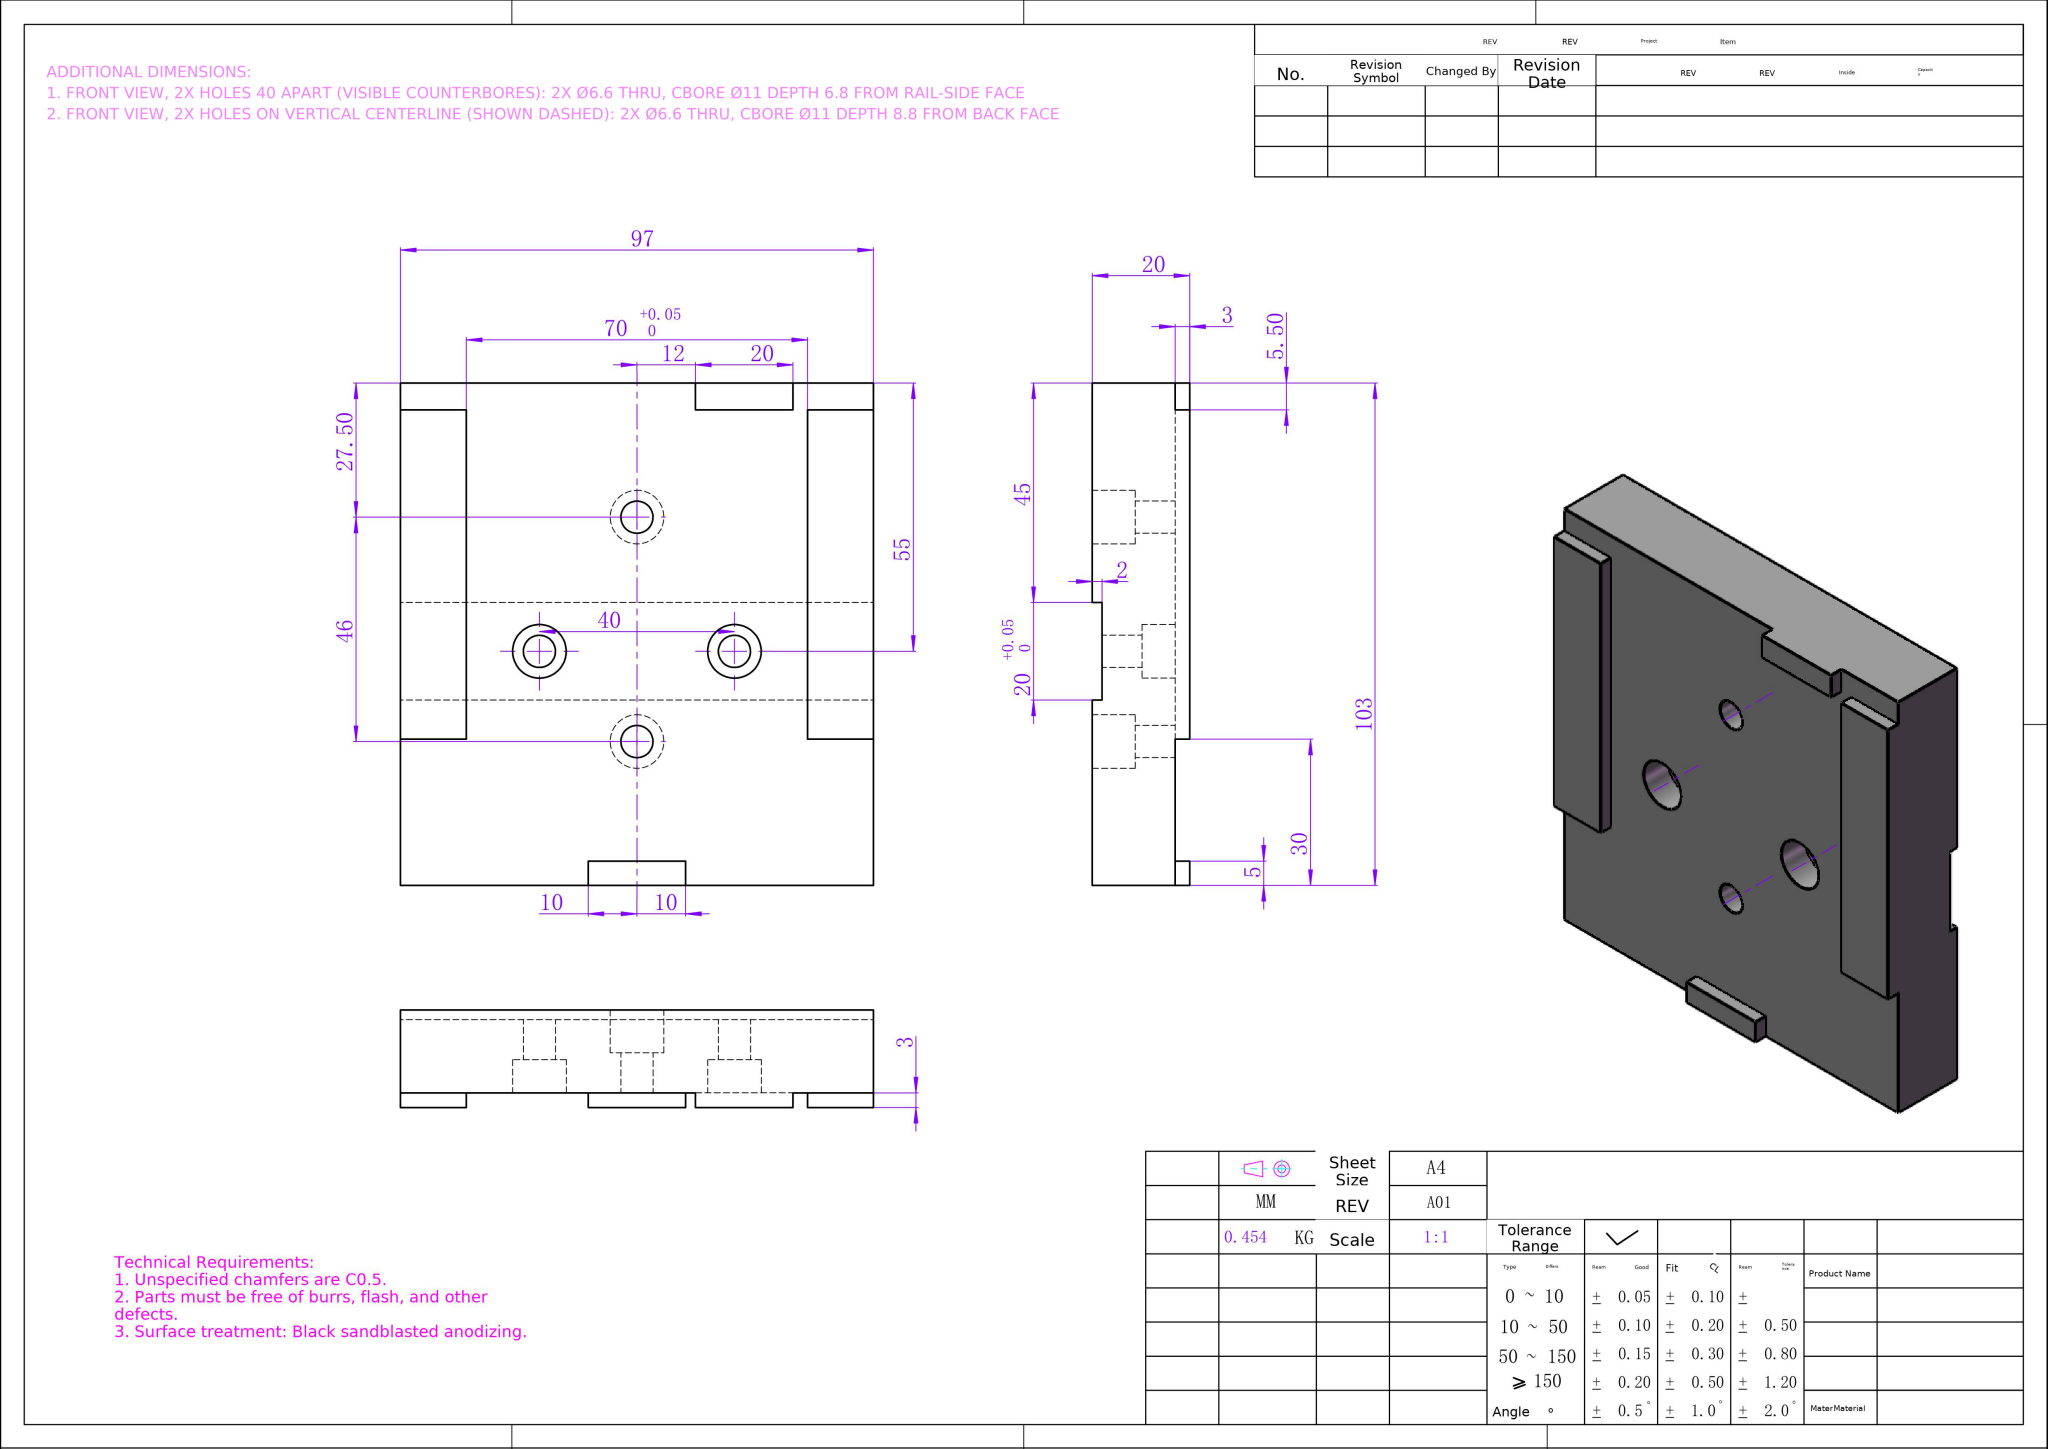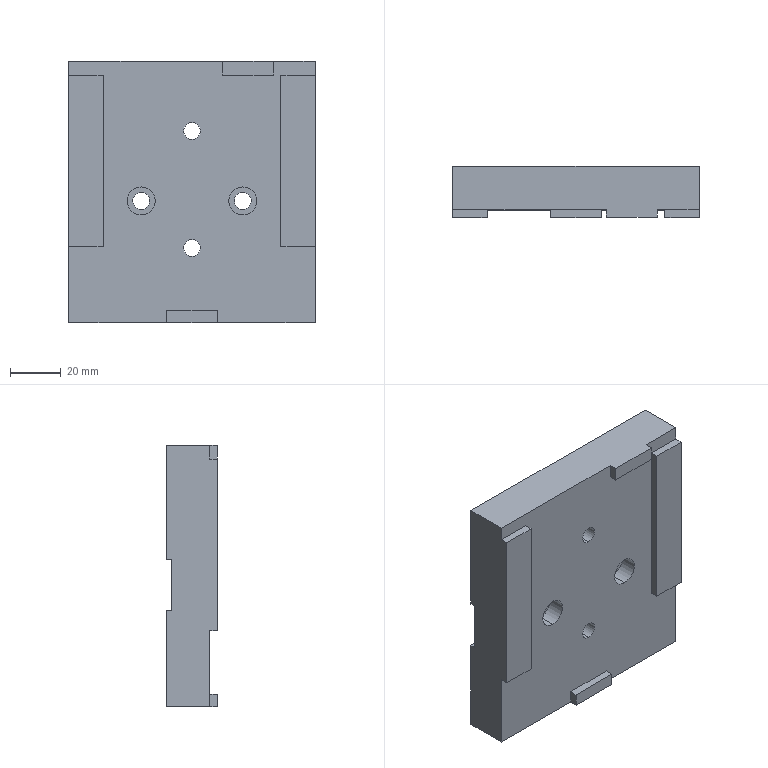Part | NX | mm | 1 solid | 46 faces | box 97 x 20 x 103 mm | volume 167977 mm3 | plane 30 | cylinder 16 | commonest cylinder face diameters 6.6 x8 11 x8